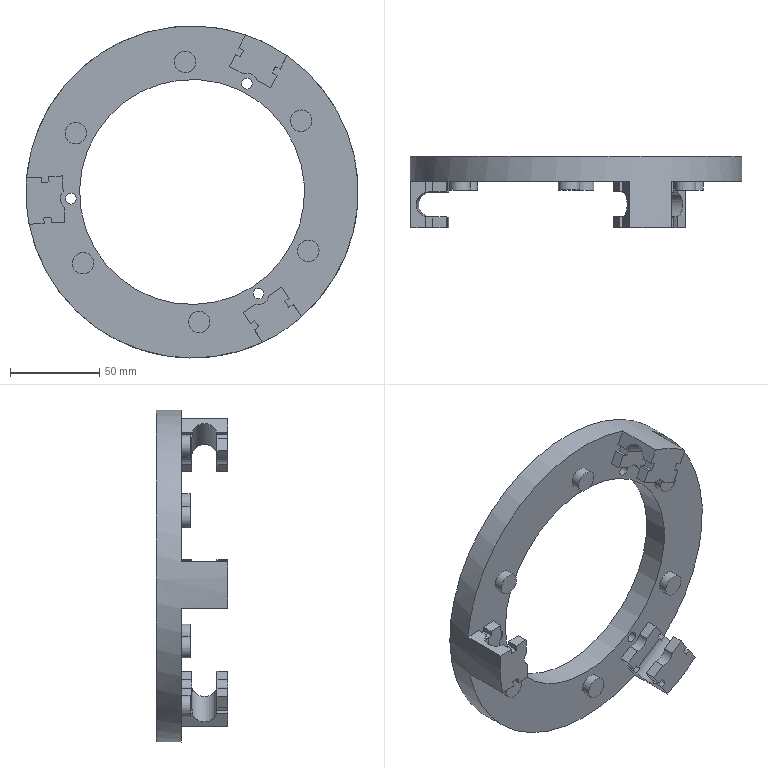Component | NX | CLUTCH_PRESSURE_PLATE | 1 solid | 103 faces | volume 231629 mm3 | plane 83 | cylinder 20 | commonest cylinder face diameters 12 x12 14 x3 6 x3 186 x1 126 x1